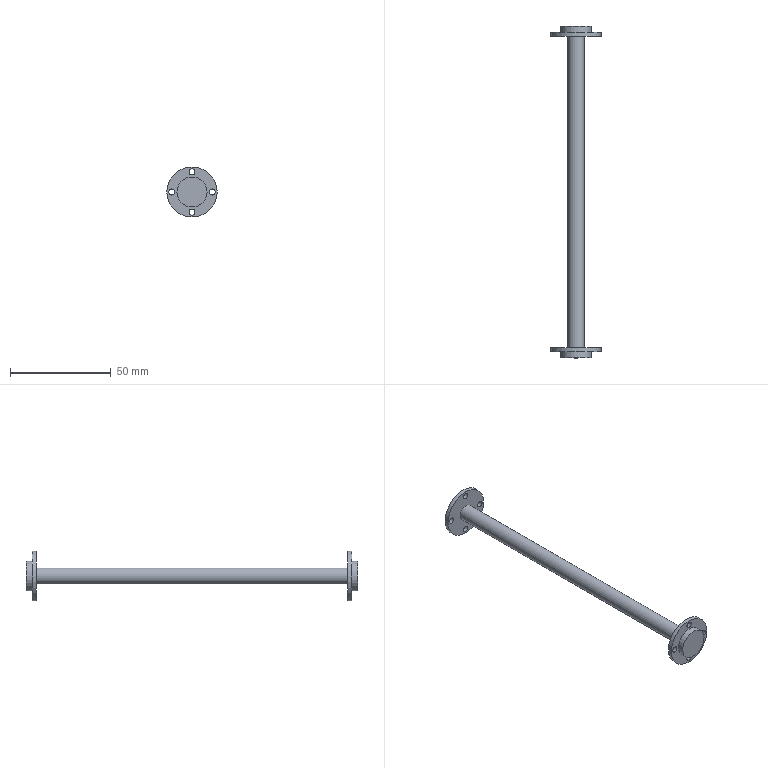Component | NX | WHEEL_AXLE | 1 solid | 19 faces | volume 10702 mm3 | cylinder 13 | plane 6 | commonest cylinder face diameters 3 x8 25 x2 15 x2 8 x1